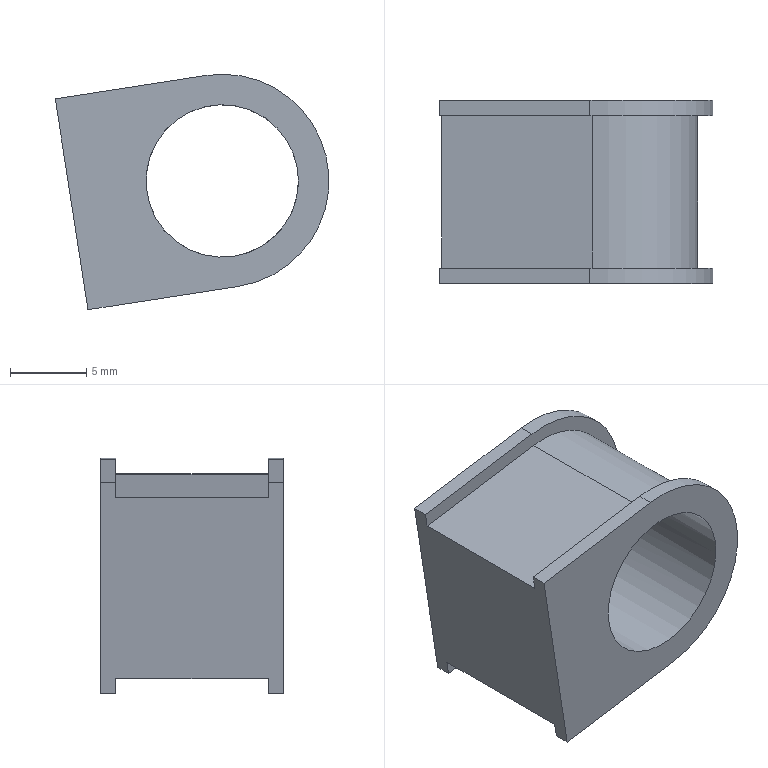Component | NX | BIG_CONN_BLOCK | 1 solid | 15 faces | volume 1257 mm3 | plane 11 | cylinder 4 | commonest cylinder face diameters 14 x2 12 x1 10 x1